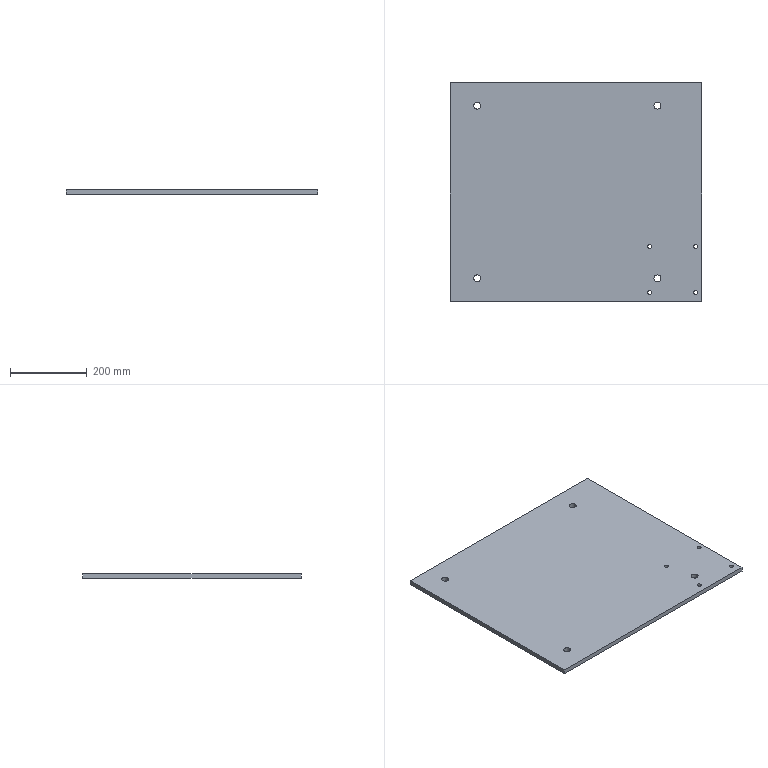Component | SolidWorks | CSFA2082 073-1 | 1 solid | 22 faces | box 655 x 570 x 12 mm | volume 4463829 mm3 | cylinder 16 | plane 6 | commonest cylinder face diameters 10.5 x8 18 x8
build123d program:
from build123d import *

# Parameters (mm, degrees)
SKETCH1_W                        = 655
SKETCH1_H                        = 570
EXTRUDE1_DEPTH                   = 12
F_18_0_18_DIAMETER_HOLE1_D       = 18
F_18_0_18_DIAMETER_HOLE1_DEPTH   = 71
F_18_0_18_DIAMETER_HOLE1_TIP     = 5.408
F_10_5_10_5_DIAMETER_HOLE1_D     = 10.5
F_10_5_10_5_DIAMETER_HOLE1_DEPTH = 71
F_10_5_10_5_DIAMETER_HOLE1_TIP   = 3.155


with BuildPart() as part:
    # Sketch1 → Extrude1 (new body)
    with BuildSketch(Plane.XY):
        Rectangle(SKETCH1_W, SKETCH1_H)
    extrude(amount=EXTRUDE1_DEPTH)

    # 18.0 _18_ Diameter Hole1
    with Locations(Plane.XY.offset(12)):
        with Locations((-257.5, 225), (-257.5, -225), (212.5, -225), (212.5, 225)):
            Hole(F_18_0_18_DIAMETER_HOLE1_D / 2, depth=F_18_0_18_DIAMETER_HOLE1_DEPTH)
            with Locations((0, 0, -(F_18_0_18_DIAMETER_HOLE1_DEPTH + F_18_0_18_DIAMETER_HOLE1_TIP / 2))):  # 118° drill point
                Cone(0, F_18_0_18_DIAMETER_HOLE1_D / 2, F_18_0_18_DIAMETER_HOLE1_TIP, mode=Mode.SUBTRACT)

    # 10.5 _10.5_ Diameter Hole1
    with Locations(Plane.XY.offset(12)):
        with Locations((312.5, -142), (192.5, -142), (192.5, -262), (312.5, -262)):
            Hole(F_10_5_10_5_DIAMETER_HOLE1_D / 2, depth=F_10_5_10_5_DIAMETER_HOLE1_DEPTH)
            with Locations((0, 0, -(F_10_5_10_5_DIAMETER_HOLE1_DEPTH + F_10_5_10_5_DIAMETER_HOLE1_TIP / 2))):  # 118° drill point
                Cone(0, F_10_5_10_5_DIAMETER_HOLE1_D / 2, F_10_5_10_5_DIAMETER_HOLE1_TIP, mode=Mode.SUBTRACT)


solid = part.part

# Placed as in the assembly
solid = solid.moved(Location((-79.949, -16.176, 445), (0, 0, 0)))
STEP:
#1=COLOUR_RGB('',0.7922,0.8196,0.9333);
#2=FILL_AREA_STYLE_COLOUR('',#1);
#3=FILL_AREA_STYLE('',(#2));
#4=SURFACE_STYLE_FILL_AREA(#3);
#5=SURFACE_SIDE_STYLE('',(#4));
#6=SURFACE_STYLE_USAGE(.BOTH.,#5);
#7=PRESENTATION_STYLE_ASSIGNMENT((#6));
#8=CARTESIAN_POINT('',(9.362,-6.227,17.52));
#9=VERTEX_POINT('',#8);
#10=CARTESIAN_POINT('',(8.949,-6.227,17.52));
#11=VERTEX_POINT('',#10);
#12=CARTESIAN_POINT('',(9.156,-6.227,17.52));
#13=DIRECTION('',(0.,0.,-1.));
#14=DIRECTION('',(-1.,0.,0.));
#15=AXIS2_PLACEMENT_3D('',#12,#13,#14);
#16=CIRCLE('',#15,0.2067);
#17=EDGE_CURVE('',#9,#11,#16,.T.);
#18=ORIENTED_EDGE('',*,*,#17,.T.);
#19=CARTESIAN_POINT('',(8.949,-6.227,17.992));
#20=VERTEX_POINT('',#19);
#21=CARTESIAN_POINT('',(8.949,-6.227,17.992));
#22=DIRECTION('',(0.,0.,1.));
#23=VECTOR('',#22,39.37);
#24=LINE('',#21,#23);
#25=EDGE_CURVE('',#11,#20,#24,.T.);
#26=ORIENTED_EDGE('',*,*,#25,.T.);
#27=CARTESIAN_POINT('',(9.362,-6.227,17.992));
#28=VERTEX_POINT('',#27);
#29=CARTESIAN_POINT('',(9.156,-6.227,17.992));
#30=DIRECTION('',(0.,0.,1.));
#31=DIRECTION('',(1.,0.,0.));
#32=AXIS2_PLACEMENT_3D('',#29,#30,#31);
#33=CIRCLE('',#32,0.2067);
#34=EDGE_CURVE('',#20,#28,#33,.T.);
#35=ORIENTED_EDGE('',*,*,#34,.T.);
#36=CARTESIAN_POINT('',(9.362,-6.227,17.992));
#37=DIRECTION('',(0.,0.,1.));
#38=VECTOR('',#37,39.37);
#39=LINE('',#36,#38);
#40=EDGE_CURVE('',#9,#28,#39,.T.);
#41=ORIENTED_EDGE('',*,*,#40,.F.);
#42=EDGE_LOOP('',(#18,#26,#35,#41));
#43=FACE_OUTER_BOUND('',#42,.T.);
#44=CARTESIAN_POINT('',(9.156,-6.227,17.992));
#45=DIRECTION('',(0.,0.,1.));
#46=DIRECTION('',(1.,0.,0.));
#47=AXIS2_PLACEMENT_3D('',#44,#45,#46);
#48=CYLINDRICAL_SURFACE('',#47,0.2067);
#49=ADVANCED_FACE('',(#43),#48,.F.);
#50=CARTESIAN_POINT('',(4.638,-6.227,17.52));
#51=VERTEX_POINT('',#50);
#52=CARTESIAN_POINT('',(4.224,-6.227,17.52));
#53=VERTEX_POINT('',#52);
#54=CARTESIAN_POINT('',(4.431,-6.227,17.52));
#55=DIRECTION('',(0.,0.,-1.));
#56=DIRECTION('',(-1.,0.,0.));
#57=AXIS2_PLACEMENT_3D('',#54,#55,#56);
#58=CIRCLE('',#57,0.2067);
#59=EDGE_CURVE('',#51,#53,#58,.T.);
#60=ORIENTED_EDGE('',*,*,#59,.T.);
#61=CARTESIAN_POINT('',(4.224,-6.227,17.992));
#62=VERTEX_POINT('',#61);
#63=CARTESIAN_POINT('',(4.224,-6.227,17.992));
#64=DIRECTION('',(0.,0.,1.));
#65=VECTOR('',#64,39.37);
#66=LINE('',#63,#65);
#67=EDGE_CURVE('',#53,#62,#66,.T.);
#68=ORIENTED_EDGE('',*,*,#67,.T.);
#69=CARTESIAN_POINT('',(4.638,-6.227,17.992));
#70=VERTEX_POINT('',#69);
#71=CARTESIAN_POINT('',(4.431,-6.227,17.992));
#72=DIRECTION('',(0.,0.,1.));
#73=DIRECTION('',(1.,0.,0.));
#74=AXIS2_PLACEMENT_3D('',#71,#72,#73);
#75=CIRCLE('',#74,0.2067);
#76=EDGE_CURVE('',#62,#70,#75,.T.);
#77=ORIENTED_EDGE('',*,*,#76,.T.);
#78=CARTESIAN_POINT('',(4.638,-6.227,17.992));
#79=DIRECTION('',(0.,0.,1.));
#80=VECTOR('',#79,39.37);
#81=LINE('',#78,#80);
#82=EDGE_CURVE('',#51,#70,#81,.T.);
#83=ORIENTED_EDGE('',*,*,#82,.F.);
#84=EDGE_LOOP('',(#60,#68,#77,#83));
#85=FACE_OUTER_BOUND('',#84,.T.);
#86=CARTESIAN_POINT('',(4.431,-6.227,17.992));
#87=DIRECTION('',(0.,0.,1.));
#88=DIRECTION('',(1.,0.,0.));
#89=AXIS2_PLACEMENT_3D('',#86,#87,#88);
#90=CYLINDRICAL_SURFACE('',#89,0.2067);
#91=ADVANCED_FACE('',(#85),#90,.F.);
#92=CARTESIAN_POINT('',(4.638,-10.952,17.52));
#93=VERTEX_POINT('',#92);
#94=CARTESIAN_POINT('',(4.224,-10.952,17.52));
#95=VERTEX_POINT('',#94);
#96=CARTESIAN_POINT('',(4.431,-10.952,17.52));
#97=DIRECTION('',(0.,0.,-1.));
#98=DIRECTION('',(-1.,0.,0.));
#99=AXIS2_PLACEMENT_3D('',#96,#97,#98);
#100=CIRCLE('',#99,0.2067);
#101=EDGE_CURVE('',#93,#95,#100,.T.);
#102=ORIENTED_EDGE('',*,*,#101,.T.);
#103=CARTESIAN_POINT('',(4.224,-10.952,17.992));
#104=VERTEX_POINT('',#103);
#105=CARTESIAN_POINT('',(4.224,-10.952,17.992));
#106=DIRECTION('',(0.,0.,1.));
#107=VECTOR('',#106,39.37);
#108=LINE('',#105,#107);
#109=EDGE_CURVE('',#95,#104,#108,.T.);
#110=ORIENTED_EDGE('',*,*,#109,.T.);
#111=CARTESIAN_POINT('',(4.638,-10.952,17.992));
#112=VERTEX_POINT('',#111);
#113=CARTESIAN_POINT('',(4.431,-10.952,17.992));
#114=DIRECTION('',(0.,0.,1.));
#115=DIRECTION('',(1.,0.,0.));
#116=AXIS2_PLACEMENT_3D('',#113,#114,#115);
#117=CIRCLE('',#116,0.2067);
#118=EDGE_CURVE('',#104,#112,#117,.T.);
#119=ORIENTED_EDGE('',*,*,#118,.T.);
#120=CARTESIAN_POINT('',(4.638,-10.952,17.992));
#121=DIRECTION('',(0.,0.,1.));
#122=VECTOR('',#121,39.37);
#123=LINE('',#120,#122);
#124=EDGE_CURVE('',#93,#112,#123,.T.);
#125=ORIENTED_EDGE('',*,*,#124,.F.);
#126=EDGE_LOOP('',(#102,#110,#119,#125));
#127=FACE_OUTER_BOUND('',#126,.T.);
#128=CARTESIAN_POINT('',(4.431,-10.952,17.992));
#129=DIRECTION('',(0.,0.,1.));
#130=DIRECTION('',(1.,0.,0.));
#131=AXIS2_PLACEMENT_3D('',#128,#129,#130);
#132=CYLINDRICAL_SURFACE('',#131,0.2067);
#133=ADVANCED_FACE('',(#127),#132,.F.);
#134=CARTESIAN_POINT('',(9.362,-10.952,17.52));
#135=VERTEX_POINT('',#134);
#136=CARTESIAN_POINT('',(8.949,-10.952,17.52));
#137=VERTEX_POINT('',#136);
#138=CARTESIAN_POINT('',(9.156,-10.952,17.52));
#139=DIRECTION('',(0.,0.,-1.));
#140=DIRECTION('',(-1.,0.,0.));
#141=AXIS2_PLACEMENT_3D('',#138,#139,#140);
#142=CIRCLE('',#141,0.2067);
#143=EDGE_CURVE('',#135,#137,#142,.T.);
#144=ORIENTED_EDGE('',*,*,#143,.T.);
#145=CARTESIAN_POINT('',(8.949,-10.952,17.992));
#146=VERTEX_POINT('',#145);
#147=CARTESIAN_POINT('',(8.949,-10.952,17.992));
#148=DIRECTION('',(0.,0.,1.));
#149=VECTOR('',#148,39.37);
#150=LINE('',#147,#149);
#151=EDGE_CURVE('',#137,#146,#150,.T.);
#152=ORIENTED_EDGE('',*,*,#151,.T.);
#153=CARTESIAN_POINT('',(9.362,-10.952,17.992));
#154=VERTEX_POINT('',#153);
#155=CARTESIAN_POINT('',(9.156,-10.952,17.992));
#156=DIRECTION('',(0.,0.,1.));
#157=DIRECTION('',(1.,0.,0.));
#158=AXIS2_PLACEMENT_3D('',#155,#156,#157);
#159=CIRCLE('',#158,0.2067);
#160=EDGE_CURVE('',#146,#154,#159,.T.);
#161=ORIENTED_EDGE('',*,*,#160,.T.);
#162=CARTESIAN_POINT('',(9.362,-10.952,17.992));
#163=DIRECTION('',(0.,0.,1.));
#164=VECTOR('',#163,39.37);
#165=LINE('',#162,#164);
#166=EDGE_CURVE('',#135,#154,#165,.T.);
#167=ORIENTED_EDGE('',*,*,#166,.F.);
#168=EDGE_LOOP('',(#144,#152,#161,#167));
#169=FACE_OUTER_BOUND('',#168,.T.);
#170=CARTESIAN_POINT('',(9.156,-10.952,17.992));
#171=DIRECTION('',(0.,0.,1.));
#172=DIRECTION('',(1.,0.,0.));
#173=AXIS2_PLACEMENT_3D('',#170,#171,#172);
#174=CYLINDRICAL_SURFACE('',#173,0.2067);
#175=ADVANCED_FACE('',(#169),#174,.F.);
#176=CARTESIAN_POINT('',(-12.931,8.221,17.52));
#177=VERTEX_POINT('',#176);
#178=CARTESIAN_POINT('',(-13.64,8.221,17.52));
#179=VERTEX_POINT('',#178);
#180=CARTESIAN_POINT('',(-13.285,8.221,17.52));
#181=DIRECTION('',(0.,0.,-1.));
#182=DIRECTION('',(-1.,0.,0.));
#183=AXIS2_PLACEMENT_3D('',#180,#181,#182);
#184=CIRCLE('',#183,0.3543);
#185=EDGE_CURVE('',#177,#179,#184,.T.);
#186=ORIENTED_EDGE('',*,*,#185,.T.);
#187=CARTESIAN_POINT('',(-13.64,8.221,17.992));
#188=VERTEX_POINT('',#187);
#189=CARTESIAN_POINT('',(-13.64,8.221,17.992));
#190=DIRECTION('',(0.,0.,1.));
#191=VECTOR('',#190,39.37);
#192=LINE('',#189,#191);
#193=EDGE_CURVE('',#179,#188,#192,.T.);
#194=ORIENTED_EDGE('',*,*,#193,.T.);
#195=CARTESIAN_POINT('',(-12.931,8.221,17.992));
#196=VERTEX_POINT('',#195);
#197=CARTESIAN_POINT('',(-13.285,8.221,17.992));
#198=DIRECTION('',(0.,0.,1.));
#199=DIRECTION('',(1.,0.,0.));
#200=AXIS2_PLACEMENT_3D('',#197,#198,#199);
#201=CIRCLE('',#200,0.3543);
#202=EDGE_CURVE('',#188,#196,#201,.T.);
#203=ORIENTED_EDGE('',*,*,#202,.T.);
#204=CARTESIAN_POINT('',(-12.931,8.221,17.992));
#205=DIRECTION('',(0.,0.,1.));
#206=VECTOR('',#205,39.37);
#207=LINE('',#204,#206);
#208=EDGE_CURVE('',#177,#196,#207,.T.);
#209=ORIENTED_EDGE('',*,*,#208,.F.);
#210=EDGE_LOOP('',(#186,#194,#203,#209));
#211=FACE_OUTER_BOUND('',#210,.T.);
#212=CARTESIAN_POINT('',(-13.285,8.221,17.992));
#213=DIRECTION('',(0.,0.,1.));
#214=DIRECTION('',(1.,0.,0.));
#215=AXIS2_PLACEMENT_3D('',#212,#213,#214);
#216=CYLINDRICAL_SURFACE('',#215,0.3543);
#217=ADVANCED_FACE('',(#211),#216,.F.);
#218=CARTESIAN_POINT('',(-12.931,-9.495,17.52));
#219=VERTEX_POINT('',#218);
#220=CARTESIAN_POINT('',(-13.64,-9.495,17.52));
#221=VERTEX_POINT('',#220);
#222=CARTESIAN_POINT('',(-13.285,-9.495,17.52));
#223=DIRECTION('',(0.,0.,-1.));
#224=DIRECTION('',(-1.,0.,0.));
#225=AXIS2_PLACEMENT_3D('',#222,#223,#224);
#226=CIRCLE('',#225,0.3543);
#227=EDGE_CURVE('',#219,#221,#226,.T.);
#228=ORIENTED_EDGE('',*,*,#227,.T.);
#229=CARTESIAN_POINT('',(-13.64,-9.495,17.992));
#230=VERTEX_POINT('',#229);
#231=CARTESIAN_POINT('',(-13.64,-9.495,17.992));
#232=DIRECTION('',(0.,0.,1.));
#233=VECTOR('',#232,39.37);
#234=LINE('',#231,#233);
#235=EDGE_CURVE('',#221,#230,#234,.T.);
#236=ORIENTED_EDGE('',*,*,#235,.T.);
#237=CARTESIAN_POINT('',(-12.931,-9.495,17.992));
#238=VERTEX_POINT('',#237);
#239=CARTESIAN_POINT('',(-13.285,-9.495,17.992));
#240=DIRECTION('',(0.,0.,1.));
#241=DIRECTION('',(1.,0.,0.));
#242=AXIS2_PLACEMENT_3D('',#239,#240,#241);
#243=CIRCLE('',#242,0.3543);
#244=EDGE_CURVE('',#230,#238,#243,.T.);
#245=ORIENTED_EDGE('',*,*,#244,.T.);
#246=CARTESIAN_POINT('',(-12.931,-9.495,17.992));
#247=DIRECTION('',(0.,0.,1.));
#248=VECTOR('',#247,39.37);
#249=LINE('',#246,#248);
#250=EDGE_CURVE('',#219,#238,#249,.T.);
#251=ORIENTED_EDGE('',*,*,#250,.F.);
#252=EDGE_LOOP('',(#228,#236,#245,#251));
#253=FACE_OUTER_BOUND('',#252,.T.);
#254=CARTESIAN_POINT('',(-13.285,-9.495,17.992));
#255=DIRECTION('',(0.,0.,1.));
#256=DIRECTION('',(1.,0.,0.));
#257=AXIS2_PLACEMENT_3D('',#254,#255,#256);
#258=CYLINDRICAL_SURFACE('',#257,0.3543);
#259=ADVANCED_FACE('',(#253),#258,.F.);
#260=CARTESIAN_POINT('',(5.573,-9.495,17.52));
#261=VERTEX_POINT('',#260);
#262=CARTESIAN_POINT('',(4.864,-9.495,17.52));
#263=VERTEX_POINT('',#262);
#264=CARTESIAN_POINT('',(5.219,-9.495,17.52));
#265=DIRECTION('',(0.,0.,-1.));
#266=DIRECTION('',(-1.,0.,0.));
#267=AXIS2_PLACEMENT_3D('',#264,#265,#266);
#268=CIRCLE('',#267,0.3543);
#269=EDGE_CURVE('',#261,#263,#268,.T.);
#270=ORIENTED_EDGE('',*,*,#269,.T.);
#271=CARTESIAN_POINT('',(4.864,-9.495,17.992));
#272=VERTEX_POINT('',#271);
#273=CARTESIAN_POINT('',(4.864,-9.495,17.992));
#274=DIRECTION('',(0.,0.,1.));
#275=VECTOR('',#274,39.37);
#276=LINE('',#273,#275);
#277=EDGE_CURVE('',#263,#272,#276,.T.);
#278=ORIENTED_EDGE('',*,*,#277,.T.);
#279=CARTESIAN_POINT('',(5.573,-9.495,17.992));
#280=VERTEX_POINT('',#279);
#281=CARTESIAN_POINT('',(5.219,-9.495,17.992));
#282=DIRECTION('',(0.,0.,1.));
#283=DIRECTION('',(1.,0.,0.));
#284=AXIS2_PLACEMENT_3D('',#281,#282,#283);
#285=CIRCLE('',#284,0.3543);
#286=EDGE_CURVE('',#272,#280,#285,.T.);
#287=ORIENTED_EDGE('',*,*,#286,.T.);
#288=CARTESIAN_POINT('',(5.573,-9.495,17.992));
#289=DIRECTION('',(0.,0.,1.));
#290=VECTOR('',#289,39.37);
#291=LINE('',#288,#290);
#292=EDGE_CURVE('',#261,#280,#291,.T.);
#293=ORIENTED_EDGE('',*,*,#292,.F.);
#294=EDGE_LOOP('',(#270,#278,#287,#293));
#295=FACE_OUTER_BOUND('',#294,.T.);
#296=CARTESIAN_POINT('',(5.219,-9.495,17.992));
#297=DIRECTION('',(0.,0.,1.));
#298=DIRECTION('',(1.,0.,0.));
#299=AXIS2_PLACEMENT_3D('',#296,#297,#298);
#300=CYLINDRICAL_SURFACE('',#299,0.3543);
#301=ADVANCED_FACE('',(#295),#300,.F.);
#302=CARTESIAN_POINT('',(5.573,8.221,17.52));
#303=VERTEX_POINT('',#302);
#304=CARTESIAN_POINT('',(4.864,8.221,17.52));
#305=VERTEX_POINT('',#304);
#306=CARTESIAN_POINT('',(5.219,8.221,17.52));
#307=DIRECTION('',(0.,0.,-1.));
#308=DIRECTION('',(-1.,0.,0.));
#309=AXIS2_PLACEMENT_3D('',#306,#307,#308);
#310=CIRCLE('',#309,0.3543);
#311=EDGE_CURVE('',#303,#305,#310,.T.);
#312=ORIENTED_EDGE('',*,*,#311,.T.);
#313=CARTESIAN_POINT('',(4.864,8.221,17.992));
#314=VERTEX_POINT('',#313);
#315=CARTESIAN_POINT('',(4.864,8.221,17.992));
#316=DIRECTION('',(0.,0.,1.));
#317=VECTOR('',#316,39.37);
#318=LINE('',#315,#317);
#319=EDGE_CURVE('',#305,#314,#318,.T.);
#320=ORIENTED_EDGE('',*,*,#319,.T.);
#321=CARTESIAN_POINT('',(5.573,8.221,17.992));
#322=VERTEX_POINT('',#321);
#323=CARTESIAN_POINT('',(5.219,8.221,17.992));
#324=DIRECTION('',(0.,0.,1.));
#325=DIRECTION('',(1.,0.,0.));
#326=AXIS2_PLACEMENT_3D('',#323,#324,#325);
#327=CIRCLE('',#326,0.3543);
#328=EDGE_CURVE('',#314,#322,#327,.T.);
#329=ORIENTED_EDGE('',*,*,#328,.T.);
#330=CARTESIAN_POINT('',(5.573,8.221,17.992));
#331=DIRECTION('',(0.,0.,1.));
#332=VECTOR('',#331,39.37);
#333=LINE('',#330,#332);
#334=EDGE_CURVE('',#303,#322,#333,.T.);
#335=ORIENTED_EDGE('',*,*,#334,.F.);
#336=EDGE_LOOP('',(#312,#320,#329,#335));
#337=FACE_OUTER_BOUND('',#336,.T.);
#338=CARTESIAN_POINT('',(5.219,8.221,17.992));
#339=DIRECTION('',(0.,0.,1.));
#340=DIRECTION('',(1.,0.,0.));
#341=AXIS2_PLACEMENT_3D('',#338,#339,#340);
#342=CYLINDRICAL_SURFACE('',#341,0.3543);
#343=ADVANCED_FACE('',(#337),#342,.F.);
#344=CARTESIAN_POINT('',(9.746,-11.857,17.52));
#345=VERTEX_POINT('',#344);
#346=CARTESIAN_POINT('',(9.746,10.584,17.52));
#347=VERTEX_POINT('',#346);
#348=CARTESIAN_POINT('',(9.746,-11.857,17.52));
#349=DIRECTION('',(0.,1.,0.));
#350=VECTOR('',#349,39.37);
#351=LINE('',#348,#350);
#352=EDGE_CURVE('',#345,#347,#351,.T.);
#353=ORIENTED_EDGE('',*,*,#352,.T.);
#354=CARTESIAN_POINT('',(9.746,10.584,17.992));
#355=VERTEX_POINT('',#354);
#356=CARTESIAN_POINT('',(9.746,10.584,17.992));
#357=DIRECTION('',(0.,0.,-1.));
#358=VECTOR('',#357,39.37);
#359=LINE('',#356,#358);
#360=EDGE_CURVE('',#355,#347,#359,.T.);
#361=ORIENTED_EDGE('',*,*,#360,.F.);
#362=CARTESIAN_POINT('',(9.746,-11.857,17.992));
#363=VERTEX_POINT('',#362);
#364=CARTESIAN_POINT('',(9.746,-11.857,17.992));
#365=DIRECTION('',(0.,1.,0.));
#366=VECTOR('',#365,39.37);
#367=LINE('',#364,#366);
#368=EDGE_CURVE('',#363,#355,#367,.T.);
#369=ORIENTED_EDGE('',*,*,#368,.F.);
#370=CARTESIAN_POINT('',(9.746,-11.857,17.992));
#371=DIRECTION('',(0.,0.,-1.));
#372=VECTOR('',#371,39.37);
#373=LINE('',#370,#372);
#374=EDGE_CURVE('',#363,#345,#373,.T.);
#375=ORIENTED_EDGE('',*,*,#374,.T.);
#376=EDGE_LOOP('',(#353,#361,#369,#375));
#377=FACE_OUTER_BOUND('',#376,.T.);
#378=CARTESIAN_POINT('',(9.746,-11.857,17.992));
#379=DIRECTION('',(-1.,0.,0.));
#380=DIRECTION('',(0.,0.,1.));
#381=AXIS2_PLACEMENT_3D('',#378,#379,#380);
#382=PLANE('',#381);
#383=ADVANCED_FACE('',(#377),#382,.F.);
#384=CARTESIAN_POINT('',(-16.041,10.584,17.52));
#385=VERTEX_POINT('',#384);
#386=CARTESIAN_POINT('',(-16.041,10.584,17.52));
#387=DIRECTION('',(-1.,0.,0.));
#388=VECTOR('',#387,39.37);
#389=LINE('',#386,#388);
#390=EDGE_CURVE('',#347,#385,#389,.T.);
#391=ORIENTED_EDGE('',*,*,#390,.T.);
#392=CARTESIAN_POINT('',(-16.041,10.584,17.992));
#393=VERTEX_POINT('',#392);
#394=CARTESIAN_POINT('',(-16.041,10.584,17.992));
#395=DIRECTION('',(0.,0.,-1.));
#396=VECTOR('',#395,39.37);
#397=LINE('',#394,#396);
#398=EDGE_CURVE('',#393,#385,#397,.T.);
#399=ORIENTED_EDGE('',*,*,#398,.F.);
#400=CARTESIAN_POINT('',(-16.041,10.584,17.992));
#401=DIRECTION('',(-1.,0.,0.));
#402=VECTOR('',#401,39.37);
#403=LINE('',#400,#402);
#404=EDGE_CURVE('',#355,#393,#403,.T.);
#405=ORIENTED_EDGE('',*,*,#404,.F.);
#406=ORIENTED_EDGE('',*,*,#360,.T.);
#407=EDGE_LOOP('',(#391,#399,#405,#406));
#408=FACE_OUTER_BOUND('',#407,.T.);
#409=CARTESIAN_POINT('',(-16.041,10.584,17.992));
#410=DIRECTION('',(0.,-1.,0.));
#411=DIRECTION('',(0.,0.,-1.));
#412=AXIS2_PLACEMENT_3D('',#409,#410,#411);
#413=PLANE('',#412);
#414=ADVANCED_FACE('',(#408),#413,.F.);
#415=CARTESIAN_POINT('',(-16.041,-11.857,17.52));
#416=VERTEX_POINT('',#415);
#417=CARTESIAN_POINT('',(-16.041,-11.857,17.52));
#418=DIRECTION('',(0.,-1.,0.));
#419=VECTOR('',#418,39.37);
#420=LINE('',#417,#419);
#421=EDGE_CURVE('',#385,#416,#420,.T.);
#422=ORIENTED_EDGE('',*,*,#421,.T.);
#423=CARTESIAN_POINT('',(-16.041,-11.857,17.992));
#424=VERTEX_POINT('',#423);
#425=CARTESIAN_POINT('',(-16.041,-11.857,17.992));
#426=DIRECTION('',(0.,0.,-1.));
#427=VECTOR('',#426,39.37);
#428=LINE('',#425,#427);
#429=EDGE_CURVE('',#424,#416,#428,.T.);
#430=ORIENTED_EDGE('',*,*,#429,.F.);
#431=CARTESIAN_POINT('',(-16.041,-11.857,17.992));
#432=DIRECTION('',(0.,-1.,0.));
#433=VECTOR('',#432,39.37);
#434=LINE('',#431,#433);
#435=EDGE_CURVE('',#393,#424,#434,.T.);
#436=ORIENTED_EDGE('',*,*,#435,.F.);
#437=ORIENTED_EDGE('',*,*,#398,.T.);
#438=EDGE_LOOP('',(#422,#430,#436,#437));
#439=FACE_OUTER_BOUND('',#438,.T.);
#440=CARTESIAN_POINT('',(-16.041,-11.857,17.992));
#441=DIRECTION('',(1.,0.,0.));
#442=DIRECTION('',(0.,0.,-1.));
#443=AXIS2_PLACEMENT_3D('',#440,#441,#442);
#444=PLANE('',#443);
#445=ADVANCED_FACE('',(#439),#444,.F.);
#446=CARTESIAN_POINT('',(-16.041,-11.857,17.52));
#447=DIRECTION('',(1.,0.,0.));
#448=VECTOR('',#447,39.37);
#449=LINE('',#446,#448);
#450=EDGE_CURVE('',#416,#345,#449,.T.);
#451=ORIENTED_EDGE('',*,*,#450,.T.);
#452=ORIENTED_EDGE('',*,*,#374,.F.);
#453=CARTESIAN_POINT('',(-16.041,-11.857,17.992));
#454=DIRECTION('',(1.,0.,0.));
#455=VECTOR('',#454,39.37);
#456=LINE('',#453,#455);
#457=EDGE_CURVE('',#424,#363,#456,.T.);
#458=ORIENTED_EDGE('',*,*,#457,.F.);
#459=ORIENTED_EDGE('',*,*,#429,.T.);
#460=EDGE_LOOP('',(#451,#452,#458,#459));
#461=FACE_OUTER_BOUND('',#460,.T.);
#462=CARTESIAN_POINT('',(-16.041,-11.857,17.992));
#463=DIRECTION('',(0.,1.,0.));
#464=DIRECTION('',(0.,0.,1.));
#465=AXIS2_PLACEMENT_3D('',#462,#463,#464);
#466=PLANE('',#465);
#467=ADVANCED_FACE('',(#461),#466,.F.);
#468=CARTESIAN_POINT('',(9.156,-6.227,17.992));
#469=DIRECTION('',(0.,0.,1.));
#470=DIRECTION('',(1.,0.,0.));
#471=AXIS2_PLACEMENT_3D('',#468,#469,#470);
#472=CIRCLE('',#471,0.2067);
#473=EDGE_CURVE('',#28,#20,#472,.T.);
#474=ORIENTED_EDGE('',*,*,#473,.F.);
#475=ORIENTED_EDGE('',*,*,#34,.F.);
#476=EDGE_LOOP('',(#474,#475));
#477=FACE_BOUND('',#476,.T.);
#478=CARTESIAN_POINT('',(4.431,-6.227,17.992));
#479=DIRECTION('',(0.,0.,1.));
#480=DIRECTION('',(1.,0.,0.));
#481=AXIS2_PLACEMENT_3D('',#478,#479,#480);
#482=CIRCLE('',#481,0.2067);
#483=EDGE_CURVE('',#70,#62,#482,.T.);
#484=ORIENTED_EDGE('',*,*,#483,.F.);
#485=ORIENTED_EDGE('',*,*,#76,.F.);
#486=EDGE_LOOP('',(#484,#485));
#487=FACE_BOUND('',#486,.T.);
#488=CARTESIAN_POINT('',(4.431,-10.952,17.992));
#489=DIRECTION('',(0.,0.,1.));
#490=DIRECTION('',(1.,0.,0.));
#491=AXIS2_PLACEMENT_3D('',#488,#489,#490);
#492=CIRCLE('',#491,0.2067);
#493=EDGE_CURVE('',#112,#104,#492,.T.);
#494=ORIENTED_EDGE('',*,*,#493,.F.);
#495=ORIENTED_EDGE('',*,*,#118,.F.);
#496=EDGE_LOOP('',(#494,#495));
#497=FACE_BOUND('',#496,.T.);
#498=CARTESIAN_POINT('',(9.156,-10.952,17.992));
#499=DIRECTION('',(0.,0.,1.));
#500=DIRECTION('',(1.,0.,0.));
#501=AXIS2_PLACEMENT_3D('',#498,#499,#500);
#502=CIRCLE('',#501,0.2067);
#503=EDGE_CURVE('',#154,#146,#502,.T.);
#504=ORIENTED_EDGE('',*,*,#503,.F.);
#505=ORIENTED_EDGE('',*,*,#160,.F.);
#506=EDGE_LOOP('',(#504,#505));
#507=FACE_BOUND('',#506,.T.);
#508=CARTESIAN_POINT('',(-13.285,8.221,17.992));
#509=DIRECTION('',(0.,0.,1.));
#510=DIRECTION('',(1.,0.,0.));
#511=AXIS2_PLACEMENT_3D('',#508,#509,#510);
#512=CIRCLE('',#511,0.3543);
#513=EDGE_CURVE('',#196,#188,#512,.T.);
#514=ORIENTED_EDGE('',*,*,#513,.F.);
#515=ORIENTED_EDGE('',*,*,#202,.F.);
#516=EDGE_LOOP('',(#514,#515));
#517=FACE_BOUND('',#516,.T.);
#518=CARTESIAN_POINT('',(-13.285,-9.495,17.992));
#519=DIRECTION('',(0.,0.,1.));
#520=DIRECTION('',(1.,0.,0.));
#521=AXIS2_PLACEMENT_3D('',#518,#519,#520);
#522=CIRCLE('',#521,0.3543);
#523=EDGE_CURVE('',#238,#230,#522,.T.);
#524=ORIENTED_EDGE('',*,*,#523,.F.);
#525=ORIENTED_EDGE('',*,*,#244,.F.);
#526=EDGE_LOOP('',(#524,#525));
#527=FACE_BOUND('',#526,.T.);
#528=CARTESIAN_POINT('',(5.219,-9.495,17.992));
#529=DIRECTION('',(0.,0.,1.));
#530=DIRECTION('',(1.,0.,0.));
#531=AXIS2_PLACEMENT_3D('',#528,#529,#530);
#532=CIRCLE('',#531,0.3543);
#533=EDGE_CURVE('',#280,#272,#532,.T.);
#534=ORIENTED_EDGE('',*,*,#533,.F.);
#535=ORIENTED_EDGE('',*,*,#286,.F.);
#536=EDGE_LOOP('',(#534,#535));
#537=FACE_BOUND('',#536,.T.);
#538=CARTESIAN_POINT('',(5.219,8.221,17.992));
#539=DIRECTION('',(0.,0.,1.));
#540=DIRECTION('',(1.,0.,0.));
#541=AXIS2_PLACEMENT_3D('',#538,#539,#540);
#542=CIRCLE('',#541,0.3543);
#543=EDGE_CURVE('',#322,#314,#542,.T.);
#544=ORIENTED_EDGE('',*,*,#543,.F.);
#545=ORIENTED_EDGE('',*,*,#328,.F.);
#546=EDGE_LOOP('',(#544,#545));
#547=FACE_BOUND('',#546,.T.);
#548=ORIENTED_EDGE('',*,*,#368,.T.);
#549=ORIENTED_EDGE('',*,*,#404,.T.);
#550=ORIENTED_EDGE('',*,*,#435,.T.);
#551=ORIENTED_EDGE('',*,*,#457,.T.);
#552=EDGE_LOOP('',(#548,#549,#550,#551));
#553=FACE_OUTER_BOUND('',#552,.T.);
#554=CARTESIAN_POINT('',(9.746,10.584,17.992));
#555=DIRECTION('',(0.,0.,-1.));
#556=DIRECTION('',(-1.,0.,0.));
#557=AXIS2_PLACEMENT_3D('',#554,#555,#556);
#558=PLANE('',#557);
#559=ADVANCED_FACE('',(#477,#487,#497,#507,#517,#527,#537,#547,#553),#558,.F.);
#560=ORIENTED_EDGE('',*,*,#17,.F.);
#561=CARTESIAN_POINT('',(9.156,-6.227,17.52));
#562=DIRECTION('',(0.,0.,-1.));
#563=DIRECTION('',(-1.,0.,0.));
#564=AXIS2_PLACEMENT_3D('',#561,#562,#563);
#565=CIRCLE('',#564,0.2067);
#566=EDGE_CURVE('',#11,#9,#565,.T.);
#567=ORIENTED_EDGE('',*,*,#566,.F.);
#568=EDGE_LOOP('',(#560,#567));
#569=FACE_BOUND('',#568,.T.);
#570=ORIENTED_EDGE('',*,*,#59,.F.);
#571=CARTESIAN_POINT('',(4.431,-6.227,17.52));
#572=DIRECTION('',(0.,0.,-1.));
#573=DIRECTION('',(-1.,0.,0.));
#574=AXIS2_PLACEMENT_3D('',#571,#572,#573);
#575=CIRCLE('',#574,0.2067);
#576=EDGE_CURVE('',#53,#51,#575,.T.);
#577=ORIENTED_EDGE('',*,*,#576,.F.);
#578=EDGE_LOOP('',(#570,#577));
#579=FACE_BOUND('',#578,.T.);
#580=ORIENTED_EDGE('',*,*,#101,.F.);
#581=CARTESIAN_POINT('',(4.431,-10.952,17.52));
#582=DIRECTION('',(0.,0.,-1.));
#583=DIRECTION('',(-1.,0.,0.));
#584=AXIS2_PLACEMENT_3D('',#581,#582,#583);
#585=CIRCLE('',#584,0.2067);
#586=EDGE_CURVE('',#95,#93,#585,.T.);
#587=ORIENTED_EDGE('',*,*,#586,.F.);
#588=EDGE_LOOP('',(#580,#587));
#589=FACE_BOUND('',#588,.T.);
#590=ORIENTED_EDGE('',*,*,#143,.F.);
#591=CARTESIAN_POINT('',(9.156,-10.952,17.52));
#592=DIRECTION('',(0.,0.,-1.));
#593=DIRECTION('',(-1.,0.,0.));
#594=AXIS2_PLACEMENT_3D('',#591,#592,#593);
#595=CIRCLE('',#594,0.2067);
#596=EDGE_CURVE('',#137,#135,#595,.T.);
#597=ORIENTED_EDGE('',*,*,#596,.F.);
#598=EDGE_LOOP('',(#590,#597));
#599=FACE_BOUND('',#598,.T.);
#600=ORIENTED_EDGE('',*,*,#185,.F.);
#601=CARTESIAN_POINT('',(-13.285,8.221,17.52));
#602=DIRECTION('',(0.,0.,-1.));
#603=DIRECTION('',(-1.,0.,0.));
#604=AXIS2_PLACEMENT_3D('',#601,#602,#603);
#605=CIRCLE('',#604,0.3543);
#606=EDGE_CURVE('',#179,#177,#605,.T.);
#607=ORIENTED_EDGE('',*,*,#606,.F.);
#608=EDGE_LOOP('',(#600,#607));
#609=FACE_BOUND('',#608,.T.);
#610=ORIENTED_EDGE('',*,*,#227,.F.);
#611=CARTESIAN_POINT('',(-13.285,-9.495,17.52));
#612=DIRECTION('',(0.,0.,-1.));
#613=DIRECTION('',(-1.,0.,0.));
#614=AXIS2_PLACEMENT_3D('',#611,#612,#613);
#615=CIRCLE('',#614,0.3543);
#616=EDGE_CURVE('',#221,#219,#615,.T.);
#617=ORIENTED_EDGE('',*,*,#616,.F.);
#618=EDGE_LOOP('',(#610,#617));
#619=FACE_BOUND('',#618,.T.);
#620=ORIENTED_EDGE('',*,*,#269,.F.);
#621=CARTESIAN_POINT('',(5.219,-9.495,17.52));
#622=DIRECTION('',(0.,0.,-1.));
#623=DIRECTION('',(-1.,0.,0.));
#624=AXIS2_PLACEMENT_3D('',#621,#622,#623);
#625=CIRCLE('',#624,0.3543);
#626=EDGE_CURVE('',#263,#261,#625,.T.);
#627=ORIENTED_EDGE('',*,*,#626,.F.);
#628=EDGE_LOOP('',(#620,#627));
#629=FACE_BOUND('',#628,.T.);
#630=ORIENTED_EDGE('',*,*,#311,.F.);
#631=CARTESIAN_POINT('',(5.219,8.221,17.52));
#632=DIRECTION('',(0.,0.,-1.));
#633=DIRECTION('',(-1.,0.,0.));
#634=AXIS2_PLACEMENT_3D('',#631,#632,#633);
#635=CIRCLE('',#634,0.3543);
#636=EDGE_CURVE('',#305,#303,#635,.T.);
#637=ORIENTED_EDGE('',*,*,#636,.F.);
#638=EDGE_LOOP('',(#630,#637));
#639=FACE_BOUND('',#638,.T.);
#640=ORIENTED_EDGE('',*,*,#352,.F.);
#641=ORIENTED_EDGE('',*,*,#450,.F.);
#642=ORIENTED_EDGE('',*,*,#421,.F.);
#643=ORIENTED_EDGE('',*,*,#390,.F.);
#644=EDGE_LOOP('',(#640,#641,#642,#643));
#645=FACE_OUTER_BOUND('',#644,.T.);
#646=CARTESIAN_POINT('',(9.746,10.584,17.52));
#647=DIRECTION('',(0.,0.,-1.));
#648=DIRECTION('',(-1.,0.,0.));
#649=AXIS2_PLACEMENT_3D('',#646,#647,#648);
#650=PLANE('',#649);
#651=ADVANCED_FACE('',(#569,#579,#589,#599,#609,#619,#629,#639,#645),#650,.T.);
#652=ORIENTED_EDGE('',*,*,#319,.F.);
#653=ORIENTED_EDGE('',*,*,#636,.T.);
#654=ORIENTED_EDGE('',*,*,#334,.T.);
#655=ORIENTED_EDGE('',*,*,#543,.T.);
#656=EDGE_LOOP('',(#652,#653,#654,#655));
#657=FACE_OUTER_BOUND('',#656,.T.);
#658=CARTESIAN_POINT('',(5.219,8.221,17.992));
#659=DIRECTION('',(0.,0.,1.));
#660=DIRECTION('',(1.,0.,0.));
#661=AXIS2_PLACEMENT_3D('',#658,#659,#660);
#662=CYLINDRICAL_SURFACE('',#661,0.3543);
#663=ADVANCED_FACE('',(#657),#662,.F.);
#664=ORIENTED_EDGE('',*,*,#277,.F.);
#665=ORIENTED_EDGE('',*,*,#626,.T.);
#666=ORIENTED_EDGE('',*,*,#292,.T.);
#667=ORIENTED_EDGE('',*,*,#533,.T.);
#668=EDGE_LOOP('',(#664,#665,#666,#667));
#669=FACE_OUTER_BOUND('',#668,.T.);
#670=CARTESIAN_POINT('',(5.219,-9.495,17.992));
#671=DIRECTION('',(0.,0.,1.));
#672=DIRECTION('',(1.,0.,0.));
#673=AXIS2_PLACEMENT_3D('',#670,#671,#672);
#674=CYLINDRICAL_SURFACE('',#673,0.3543);
#675=ADVANCED_FACE('',(#669),#674,.F.);
#676=ORIENTED_EDGE('',*,*,#235,.F.);
#677=ORIENTED_EDGE('',*,*,#616,.T.);
#678=ORIENTED_EDGE('',*,*,#250,.T.);
#679=ORIENTED_EDGE('',*,*,#523,.T.);
#680=EDGE_LOOP('',(#676,#677,#678,#679));
#681=FACE_OUTER_BOUND('',#680,.T.);
#682=CARTESIAN_POINT('',(-13.285,-9.495,17.992));
#683=DIRECTION('',(0.,0.,1.));
#684=DIRECTION('',(1.,0.,0.));
#685=AXIS2_PLACEMENT_3D('',#682,#683,#684);
#686=CYLINDRICAL_SURFACE('',#685,0.3543);
#687=ADVANCED_FACE('',(#681),#686,.F.);
#688=ORIENTED_EDGE('',*,*,#193,.F.);
#689=ORIENTED_EDGE('',*,*,#606,.T.);
#690=ORIENTED_EDGE('',*,*,#208,.T.);
#691=ORIENTED_EDGE('',*,*,#513,.T.);
#692=EDGE_LOOP('',(#688,#689,#690,#691));
#693=FACE_OUTER_BOUND('',#692,.T.);
#694=CARTESIAN_POINT('',(-13.285,8.221,17.992));
#695=DIRECTION('',(0.,0.,1.));
#696=DIRECTION('',(1.,0.,0.));
#697=AXIS2_PLACEMENT_3D('',#694,#695,#696);
#698=CYLINDRICAL_SURFACE('',#697,0.3543);
#699=ADVANCED_FACE('',(#693),#698,.F.);
#700=ORIENTED_EDGE('',*,*,#151,.F.);
#701=ORIENTED_EDGE('',*,*,#596,.T.);
#702=ORIENTED_EDGE('',*,*,#166,.T.);
#703=ORIENTED_EDGE('',*,*,#503,.T.);
#704=EDGE_LOOP('',(#700,#701,#702,#703));
#705=FACE_OUTER_BOUND('',#704,.T.);
#706=CARTESIAN_POINT('',(9.156,-10.952,17.992));
#707=DIRECTION('',(0.,0.,1.));
#708=DIRECTION('',(1.,0.,0.));
#709=AXIS2_PLACEMENT_3D('',#706,#707,#708);
#710=CYLINDRICAL_SURFACE('',#709,0.2067);
#711=ADVANCED_FACE('',(#705),#710,.F.);
#712=ORIENTED_EDGE('',*,*,#109,.F.);
#713=ORIENTED_EDGE('',*,*,#586,.T.);
#714=ORIENTED_EDGE('',*,*,#124,.T.);
#715=ORIENTED_EDGE('',*,*,#493,.T.);
#716=EDGE_LOOP('',(#712,#713,#714,#715));
#717=FACE_OUTER_BOUND('',#716,.T.);
#718=CARTESIAN_POINT('',(4.431,-10.952,17.992));
#719=DIRECTION('',(0.,0.,1.));
#720=DIRECTION('',(1.,0.,0.));
#721=AXIS2_PLACEMENT_3D('',#718,#719,#720);
#722=CYLINDRICAL_SURFACE('',#721,0.2067);
#723=ADVANCED_FACE('',(#717),#722,.F.);
#724=ORIENTED_EDGE('',*,*,#67,.F.);
#725=ORIENTED_EDGE('',*,*,#576,.T.);
#726=ORIENTED_EDGE('',*,*,#82,.T.);
#727=ORIENTED_EDGE('',*,*,#483,.T.);
#728=EDGE_LOOP('',(#724,#725,#726,#727));
#729=FACE_OUTER_BOUND('',#728,.T.);
#730=CARTESIAN_POINT('',(4.431,-6.227,17.992));
#731=DIRECTION('',(0.,0.,1.));
#732=DIRECTION('',(1.,0.,0.));
#733=AXIS2_PLACEMENT_3D('',#730,#731,#732);
#734=CYLINDRICAL_SURFACE('',#733,0.2067);
#735=ADVANCED_FACE('',(#729),#734,.F.);
#736=ORIENTED_EDGE('',*,*,#25,.F.);
#737=ORIENTED_EDGE('',*,*,#566,.T.);
#738=ORIENTED_EDGE('',*,*,#40,.T.);
#739=ORIENTED_EDGE('',*,*,#473,.T.);
#740=EDGE_LOOP('',(#736,#737,#738,#739));
#741=FACE_OUTER_BOUND('',#740,.T.);
#742=CARTESIAN_POINT('',(9.156,-6.227,17.992));
#743=DIRECTION('',(0.,0.,1.));
#744=DIRECTION('',(1.,0.,0.));
#745=AXIS2_PLACEMENT_3D('',#742,#743,#744);
#746=CYLINDRICAL_SURFACE('',#745,0.2067);
#747=ADVANCED_FACE('',(#741),#746,.F.);
#748=CLOSED_SHELL('',(#49,#91,#133,#175,#217,#259,#301,#343,#383,#414,#445,#467,#559,#651,#663,#675,#687,#699,#711,#723,#735,#747));
#749=MANIFOLD_SOLID_BREP('',#748);
#750=STYLED_ITEM('',(#7),#749);
#751=PRESENTATION_LAYER_ASSIGNMENT('','',(#750));
#752=CARTESIAN_POINT('',(0.,0.,0.));
#753=DIRECTION('',(0.,0.,1.));
#754=DIRECTION('',(1.,0.,0.));
#755=AXIS2_PLACEMENT_3D('',#752,#753,#754);
#756=(LENGTH_UNIT()NAMED_UNIT(*)SI_UNIT($,.METRE.));
#757=LENGTH_MEASURE_WITH_UNIT(LENGTH_MEASURE(0.0254),#756);
#758=DIMENSIONAL_EXPONENTS(1.,0.,0.,0.,0.,0.,0.);
#759=(CONVERSION_BASED_UNIT('',#757)LENGTH_UNIT()NAMED_UNIT(#758));
#760=UNCERTAINTY_MEASURE_WITH_UNIT(LENGTH_MEASURE(0.00001),#759,'','');
#761=(NAMED_UNIT(*)PLANE_ANGLE_UNIT()SI_UNIT($,.RADIAN.));
#762=(NAMED_UNIT(*)SI_UNIT($,.STERADIAN.)SOLID_ANGLE_UNIT());
#763=(GEOMETRIC_REPRESENTATION_CONTEXT(3)GLOBAL_UNCERTAINTY_ASSIGNED_CONTEXT((#760))GLOBAL_UNIT_ASSIGNED_CONTEXT((#759,#761,#762))REPRESENTATION_CONTEXT('',''));
#764=ADVANCED_BREP_SHAPE_REPRESENTATION('',(#749,#755),#763);
#765=(LENGTH_UNIT()NAMED_UNIT(*)SI_UNIT($,.METRE.));
#766=LENGTH_MEASURE_WITH_UNIT(LENGTH_MEASURE(0.0254),#765);
#767=DIMENSIONAL_EXPONENTS(1.,0.,0.,0.,0.,0.,0.);
#768=(CONVERSION_BASED_UNIT('',#766)LENGTH_UNIT()NAMED_UNIT(#767));
#769=UNCERTAINTY_MEASURE_WITH_UNIT(LENGTH_MEASURE(0.00001),#768,'','');
#770=(NAMED_UNIT(*)PLANE_ANGLE_UNIT()SI_UNIT($,.RADIAN.));
#771=(NAMED_UNIT(*)SI_UNIT($,.STERADIAN.)SOLID_ANGLE_UNIT());
#772=(GEOMETRIC_REPRESENTATION_CONTEXT(3)GLOBAL_UNCERTAINTY_ASSIGNED_CONTEXT((#769))GLOBAL_UNIT_ASSIGNED_CONTEXT((#768,#770,#771))REPRESENTATION_CONTEXT('',''));
#773=MECHANICAL_DESIGN_GEOMETRIC_PRESENTATION_REPRESENTATION('',(#750),#772);